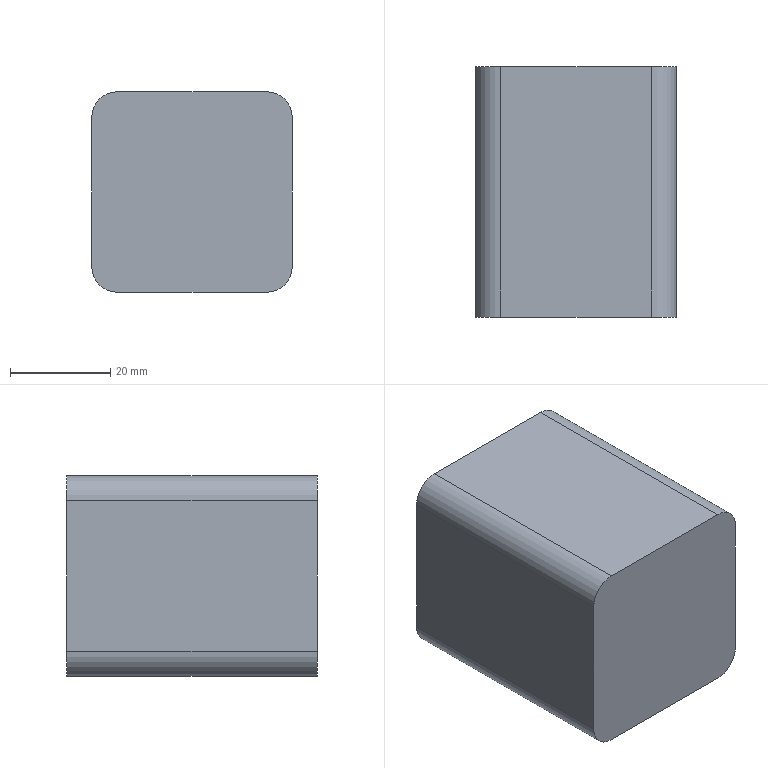Component | SolidWorks | Jig4040-50-5 | 1 solid | 10 faces | box 40 x 50 x 40 mm | volume 78927 mm3 | plane 6 | cylinder 4 | commonest cylinder face diameters 10 x4 | material Copper
build123d program:
from build123d import *

# Parameters (mm, degrees)
BOSS_EXTRUDE1_DEPTH = 50


with BuildPart() as part:
    # Sketch1 → Boss-Extrude1 (new body)
    with BuildSketch(Plane(origin=(0, 0, 0), x_dir=(1, 0, 0), z_dir=(0, 1, 0))):
        with BuildLine():
            Line((5, 0), (35, 0))
            ThreePointArc((35, 0), (38.536, 1.464), (40, 5))
            Line((40, 5), (40, 35))
            ThreePointArc((40, 35), (38.536, 38.536), (35, 40))
            Line((35, 40), (5, 40))
            ThreePointArc((5, 40), (1.464, 38.536), (0, 35))
            Line((0, 35), (0, 5))
            ThreePointArc((0, 5), (1.464, 1.464), (5, 0))
        make_face()
    extrude(amount=BOSS_EXTRUDE1_DEPTH)


solid = part.part

# Placed as in the assembly
solid = solid.moved(Location((711.992, -67.909, 2130), (0, 0, 0)))
STEP:
#1=COLOUR_RGB('',0.7922,0.8196,0.9333);
#2=FILL_AREA_STYLE_COLOUR('',#1);
#3=FILL_AREA_STYLE('',(#2));
#4=SURFACE_STYLE_FILL_AREA(#3);
#5=SURFACE_SIDE_STYLE('',(#4));
#6=SURFACE_STYLE_USAGE(.BOTH.,#5);
#7=PRESENTATION_STYLE_ASSIGNMENT((#6));
#8=CARTESIAN_POINT('',(28.031,-2.674,83.661));
#9=VERTEX_POINT('',#8);
#10=CARTESIAN_POINT('',(28.228,-2.674,83.858));
#11=VERTEX_POINT('',#10);
#12=CARTESIAN_POINT('',(28.228,-2.674,83.661));
#13=DIRECTION('',(0.,1.,0.));
#14=DIRECTION('',(0.,0.,1.));
#15=AXIS2_PLACEMENT_3D('',#12,#13,#14);
#16=CIRCLE('',#15,0.1969);
#17=EDGE_CURVE('',#9,#11,#16,.T.);
#18=ORIENTED_EDGE('',*,*,#17,.T.);
#19=CARTESIAN_POINT('',(28.228,-0.7051,83.858));
#20=VERTEX_POINT('',#19);
#21=CARTESIAN_POINT('',(28.228,-0.7051,83.858));
#22=DIRECTION('',(0.,-1.,0.));
#23=VECTOR('',#22,39.37);
#24=LINE('',#21,#23);
#25=EDGE_CURVE('',#20,#11,#24,.T.);
#26=ORIENTED_EDGE('',*,*,#25,.F.);
#27=CARTESIAN_POINT('',(28.031,-0.7051,83.661));
#28=VERTEX_POINT('',#27);
#29=CARTESIAN_POINT('',(28.228,-0.7051,83.661));
#30=DIRECTION('',(0.,1.,0.));
#31=DIRECTION('',(0.,0.,1.));
#32=AXIS2_PLACEMENT_3D('',#29,#30,#31);
#33=CIRCLE('',#32,0.1969);
#34=EDGE_CURVE('',#28,#20,#33,.T.);
#35=ORIENTED_EDGE('',*,*,#34,.F.);
#36=CARTESIAN_POINT('',(28.031,-0.7051,83.661));
#37=DIRECTION('',(0.,-1.,0.));
#38=VECTOR('',#37,39.37);
#39=LINE('',#36,#38);
#40=EDGE_CURVE('',#28,#9,#39,.T.);
#41=ORIENTED_EDGE('',*,*,#40,.T.);
#42=EDGE_LOOP('',(#18,#26,#35,#41));
#43=FACE_OUTER_BOUND('',#42,.T.);
#44=CARTESIAN_POINT('',(28.228,-0.7051,83.661));
#45=DIRECTION('',(0.,-1.,0.));
#46=DIRECTION('',(0.,0.,-1.));
#47=AXIS2_PLACEMENT_3D('',#44,#45,#46);
#48=CYLINDRICAL_SURFACE('',#47,0.1969);
#49=ADVANCED_FACE('',(#43),#48,.T.);
#50=CARTESIAN_POINT('',(29.409,-2.674,83.858));
#51=VERTEX_POINT('',#50);
#52=CARTESIAN_POINT('',(28.228,-2.674,83.858));
#53=DIRECTION('',(1.,0.,0.));
#54=VECTOR('',#53,39.37);
#55=LINE('',#52,#54);
#56=EDGE_CURVE('',#11,#51,#55,.T.);
#57=ORIENTED_EDGE('',*,*,#56,.T.);
#58=CARTESIAN_POINT('',(29.409,-0.7051,83.858));
#59=VERTEX_POINT('',#58);
#60=CARTESIAN_POINT('',(29.409,-0.7051,83.858));
#61=DIRECTION('',(0.,-1.,0.));
#62=VECTOR('',#61,39.37);
#63=LINE('',#60,#62);
#64=EDGE_CURVE('',#59,#51,#63,.T.);
#65=ORIENTED_EDGE('',*,*,#64,.F.);
#66=CARTESIAN_POINT('',(28.228,-0.7051,83.858));
#67=DIRECTION('',(1.,0.,0.));
#68=VECTOR('',#67,39.37);
#69=LINE('',#66,#68);
#70=EDGE_CURVE('',#20,#59,#69,.T.);
#71=ORIENTED_EDGE('',*,*,#70,.F.);
#72=ORIENTED_EDGE('',*,*,#25,.T.);
#73=EDGE_LOOP('',(#57,#65,#71,#72));
#74=FACE_OUTER_BOUND('',#73,.T.);
#75=CARTESIAN_POINT('',(28.228,-0.7051,83.858));
#76=DIRECTION('',(0.,0.,-1.));
#77=DIRECTION('',(-1.,0.,0.));
#78=AXIS2_PLACEMENT_3D('',#75,#76,#77);
#79=PLANE('',#78);
#80=ADVANCED_FACE('',(#74),#79,.F.);
#81=CARTESIAN_POINT('',(29.606,-2.674,83.661));
#82=VERTEX_POINT('',#81);
#83=CARTESIAN_POINT('',(29.409,-2.674,83.661));
#84=DIRECTION('',(0.,1.,0.));
#85=DIRECTION('',(0.,0.,1.));
#86=AXIS2_PLACEMENT_3D('',#83,#84,#85);
#87=CIRCLE('',#86,0.1969);
#88=EDGE_CURVE('',#51,#82,#87,.T.);
#89=ORIENTED_EDGE('',*,*,#88,.T.);
#90=CARTESIAN_POINT('',(29.606,-0.7051,83.661));
#91=VERTEX_POINT('',#90);
#92=CARTESIAN_POINT('',(29.606,-0.7051,83.661));
#93=DIRECTION('',(0.,-1.,0.));
#94=VECTOR('',#93,39.37);
#95=LINE('',#92,#94);
#96=EDGE_CURVE('',#91,#82,#95,.T.);
#97=ORIENTED_EDGE('',*,*,#96,.F.);
#98=CARTESIAN_POINT('',(29.409,-0.7051,83.661));
#99=DIRECTION('',(0.,1.,0.));
#100=DIRECTION('',(0.,0.,1.));
#101=AXIS2_PLACEMENT_3D('',#98,#99,#100);
#102=CIRCLE('',#101,0.1969);
#103=EDGE_CURVE('',#59,#91,#102,.T.);
#104=ORIENTED_EDGE('',*,*,#103,.F.);
#105=ORIENTED_EDGE('',*,*,#64,.T.);
#106=EDGE_LOOP('',(#89,#97,#104,#105));
#107=FACE_OUTER_BOUND('',#106,.T.);
#108=CARTESIAN_POINT('',(29.409,-0.7051,83.661));
#109=DIRECTION('',(0.,-1.,0.));
#110=DIRECTION('',(0.,0.,-1.));
#111=AXIS2_PLACEMENT_3D('',#108,#109,#110);
#112=CYLINDRICAL_SURFACE('',#111,0.1969);
#113=ADVANCED_FACE('',(#107),#112,.T.);
#114=CARTESIAN_POINT('',(29.606,-2.674,82.48));
#115=VERTEX_POINT('',#114);
#116=CARTESIAN_POINT('',(29.606,-2.674,83.661));
#117=DIRECTION('',(0.,0.,-1.));
#118=VECTOR('',#117,39.37);
#119=LINE('',#116,#118);
#120=EDGE_CURVE('',#82,#115,#119,.T.);
#121=ORIENTED_EDGE('',*,*,#120,.T.);
#122=CARTESIAN_POINT('',(29.606,-0.7051,82.48));
#123=VERTEX_POINT('',#122);
#124=CARTESIAN_POINT('',(29.606,-0.7051,82.48));
#125=DIRECTION('',(0.,-1.,0.));
#126=VECTOR('',#125,39.37);
#127=LINE('',#124,#126);
#128=EDGE_CURVE('',#123,#115,#127,.T.);
#129=ORIENTED_EDGE('',*,*,#128,.F.);
#130=CARTESIAN_POINT('',(29.606,-0.7051,83.661));
#131=DIRECTION('',(0.,0.,-1.));
#132=VECTOR('',#131,39.37);
#133=LINE('',#130,#132);
#134=EDGE_CURVE('',#91,#123,#133,.T.);
#135=ORIENTED_EDGE('',*,*,#134,.F.);
#136=ORIENTED_EDGE('',*,*,#96,.T.);
#137=EDGE_LOOP('',(#121,#129,#135,#136));
#138=FACE_OUTER_BOUND('',#137,.T.);
#139=CARTESIAN_POINT('',(29.606,-0.7051,83.661));
#140=DIRECTION('',(-1.,0.,0.));
#141=DIRECTION('',(0.,0.,1.));
#142=AXIS2_PLACEMENT_3D('',#139,#140,#141);
#143=PLANE('',#142);
#144=ADVANCED_FACE('',(#138),#143,.F.);
#145=CARTESIAN_POINT('',(29.409,-2.674,82.283));
#146=VERTEX_POINT('',#145);
#147=CARTESIAN_POINT('',(29.409,-2.674,82.48));
#148=DIRECTION('',(0.,1.,0.));
#149=DIRECTION('',(0.,0.,-1.));
#150=AXIS2_PLACEMENT_3D('',#147,#148,#149);
#151=CIRCLE('',#150,0.1969);
#152=EDGE_CURVE('',#115,#146,#151,.T.);
#153=ORIENTED_EDGE('',*,*,#152,.T.);
#154=CARTESIAN_POINT('',(29.409,-0.7051,82.283));
#155=VERTEX_POINT('',#154);
#156=CARTESIAN_POINT('',(29.409,-0.7051,82.283));
#157=DIRECTION('',(0.,-1.,0.));
#158=VECTOR('',#157,39.37);
#159=LINE('',#156,#158);
#160=EDGE_CURVE('',#155,#146,#159,.T.);
#161=ORIENTED_EDGE('',*,*,#160,.F.);
#162=CARTESIAN_POINT('',(29.409,-0.7051,82.48));
#163=DIRECTION('',(0.,1.,0.));
#164=DIRECTION('',(0.,0.,-1.));
#165=AXIS2_PLACEMENT_3D('',#162,#163,#164);
#166=CIRCLE('',#165,0.1969);
#167=EDGE_CURVE('',#123,#155,#166,.T.);
#168=ORIENTED_EDGE('',*,*,#167,.F.);
#169=ORIENTED_EDGE('',*,*,#128,.T.);
#170=EDGE_LOOP('',(#153,#161,#168,#169));
#171=FACE_OUTER_BOUND('',#170,.T.);
#172=CARTESIAN_POINT('',(29.409,-0.7051,82.48));
#173=DIRECTION('',(0.,-1.,0.));
#174=DIRECTION('',(0.,0.,-1.));
#175=AXIS2_PLACEMENT_3D('',#172,#173,#174);
#176=CYLINDRICAL_SURFACE('',#175,0.1969);
#177=ADVANCED_FACE('',(#171),#176,.T.);
#178=CARTESIAN_POINT('',(28.228,-2.674,82.283));
#179=VERTEX_POINT('',#178);
#180=CARTESIAN_POINT('',(28.228,-2.674,82.283));
#181=DIRECTION('',(-1.,0.,0.));
#182=VECTOR('',#181,39.37);
#183=LINE('',#180,#182);
#184=EDGE_CURVE('',#146,#179,#183,.T.);
#185=ORIENTED_EDGE('',*,*,#184,.T.);
#186=CARTESIAN_POINT('',(28.228,-0.7051,82.283));
#187=VERTEX_POINT('',#186);
#188=CARTESIAN_POINT('',(28.228,-0.7051,82.283));
#189=DIRECTION('',(0.,-1.,0.));
#190=VECTOR('',#189,39.37);
#191=LINE('',#188,#190);
#192=EDGE_CURVE('',#187,#179,#191,.T.);
#193=ORIENTED_EDGE('',*,*,#192,.F.);
#194=CARTESIAN_POINT('',(28.228,-0.7051,82.283));
#195=DIRECTION('',(-1.,0.,0.));
#196=VECTOR('',#195,39.37);
#197=LINE('',#194,#196);
#198=EDGE_CURVE('',#155,#187,#197,.T.);
#199=ORIENTED_EDGE('',*,*,#198,.F.);
#200=ORIENTED_EDGE('',*,*,#160,.T.);
#201=EDGE_LOOP('',(#185,#193,#199,#200));
#202=FACE_OUTER_BOUND('',#201,.T.);
#203=CARTESIAN_POINT('',(28.228,-0.7051,82.283));
#204=DIRECTION('',(0.,0.,1.));
#205=DIRECTION('',(1.,0.,0.));
#206=AXIS2_PLACEMENT_3D('',#203,#204,#205);
#207=PLANE('',#206);
#208=ADVANCED_FACE('',(#202),#207,.F.);
#209=CARTESIAN_POINT('',(28.031,-2.674,82.48));
#210=VERTEX_POINT('',#209);
#211=CARTESIAN_POINT('',(28.228,-2.674,82.48));
#212=DIRECTION('',(0.,1.,0.));
#213=DIRECTION('',(0.,0.,-1.));
#214=AXIS2_PLACEMENT_3D('',#211,#212,#213);
#215=CIRCLE('',#214,0.1969);
#216=EDGE_CURVE('',#179,#210,#215,.T.);
#217=ORIENTED_EDGE('',*,*,#216,.T.);
#218=CARTESIAN_POINT('',(28.031,-0.7051,82.48));
#219=VERTEX_POINT('',#218);
#220=CARTESIAN_POINT('',(28.031,-0.7051,82.48));
#221=DIRECTION('',(0.,-1.,0.));
#222=VECTOR('',#221,39.37);
#223=LINE('',#220,#222);
#224=EDGE_CURVE('',#219,#210,#223,.T.);
#225=ORIENTED_EDGE('',*,*,#224,.F.);
#226=CARTESIAN_POINT('',(28.228,-0.7051,82.48));
#227=DIRECTION('',(0.,1.,0.));
#228=DIRECTION('',(0.,0.,-1.));
#229=AXIS2_PLACEMENT_3D('',#226,#227,#228);
#230=CIRCLE('',#229,0.1969);
#231=EDGE_CURVE('',#187,#219,#230,.T.);
#232=ORIENTED_EDGE('',*,*,#231,.F.);
#233=ORIENTED_EDGE('',*,*,#192,.T.);
#234=EDGE_LOOP('',(#217,#225,#232,#233));
#235=FACE_OUTER_BOUND('',#234,.T.);
#236=CARTESIAN_POINT('',(28.228,-0.7051,82.48));
#237=DIRECTION('',(0.,-1.,0.));
#238=DIRECTION('',(0.,0.,-1.));
#239=AXIS2_PLACEMENT_3D('',#236,#237,#238);
#240=CYLINDRICAL_SURFACE('',#239,0.1969);
#241=ADVANCED_FACE('',(#235),#240,.T.);
#242=CARTESIAN_POINT('',(28.031,-2.674,83.661));
#243=DIRECTION('',(0.,0.,1.));
#244=VECTOR('',#243,39.37);
#245=LINE('',#242,#244);
#246=EDGE_CURVE('',#210,#9,#245,.T.);
#247=ORIENTED_EDGE('',*,*,#246,.T.);
#248=ORIENTED_EDGE('',*,*,#40,.F.);
#249=CARTESIAN_POINT('',(28.031,-0.7051,83.661));
#250=DIRECTION('',(0.,0.,1.));
#251=VECTOR('',#250,39.37);
#252=LINE('',#249,#251);
#253=EDGE_CURVE('',#219,#28,#252,.T.);
#254=ORIENTED_EDGE('',*,*,#253,.F.);
#255=ORIENTED_EDGE('',*,*,#224,.T.);
#256=EDGE_LOOP('',(#247,#248,#254,#255));
#257=FACE_OUTER_BOUND('',#256,.T.);
#258=CARTESIAN_POINT('',(28.031,-0.7051,83.661));
#259=DIRECTION('',(1.,0.,0.));
#260=DIRECTION('',(0.,0.,-1.));
#261=AXIS2_PLACEMENT_3D('',#258,#259,#260);
#262=PLANE('',#261);
#263=ADVANCED_FACE('',(#257),#262,.F.);
#264=ORIENTED_EDGE('',*,*,#34,.T.);
#265=ORIENTED_EDGE('',*,*,#70,.T.);
#266=ORIENTED_EDGE('',*,*,#103,.T.);
#267=ORIENTED_EDGE('',*,*,#134,.T.);
#268=ORIENTED_EDGE('',*,*,#167,.T.);
#269=ORIENTED_EDGE('',*,*,#198,.T.);
#270=ORIENTED_EDGE('',*,*,#231,.T.);
#271=ORIENTED_EDGE('',*,*,#253,.T.);
#272=EDGE_LOOP('',(#264,#265,#266,#267,#268,#269,#270,#271));
#273=FACE_OUTER_BOUND('',#272,.T.);
#274=CARTESIAN_POINT('',(28.228,-0.7051,83.661));
#275=DIRECTION('',(0.,1.,0.));
#276=DIRECTION('',(0.,0.,1.));
#277=AXIS2_PLACEMENT_3D('',#274,#275,#276);
#278=PLANE('',#277);
#279=ADVANCED_FACE('',(#273),#278,.T.);
#280=ORIENTED_EDGE('',*,*,#17,.F.);
#281=ORIENTED_EDGE('',*,*,#246,.F.);
#282=ORIENTED_EDGE('',*,*,#216,.F.);
#283=ORIENTED_EDGE('',*,*,#184,.F.);
#284=ORIENTED_EDGE('',*,*,#152,.F.);
#285=ORIENTED_EDGE('',*,*,#120,.F.);
#286=ORIENTED_EDGE('',*,*,#88,.F.);
#287=ORIENTED_EDGE('',*,*,#56,.F.);
#288=EDGE_LOOP('',(#280,#281,#282,#283,#284,#285,#286,#287));
#289=FACE_OUTER_BOUND('',#288,.T.);
#290=CARTESIAN_POINT('',(28.228,-2.674,83.661));
#291=DIRECTION('',(0.,1.,0.));
#292=DIRECTION('',(0.,0.,1.));
#293=AXIS2_PLACEMENT_3D('',#290,#291,#292);
#294=PLANE('',#293);
#295=ADVANCED_FACE('',(#289),#294,.F.);
#296=CLOSED_SHELL('',(#49,#80,#113,#144,#177,#208,#241,#263,#279,#295));
#297=MANIFOLD_SOLID_BREP('',#296);
#298=STYLED_ITEM('',(#7),#297);
#299=PRESENTATION_LAYER_ASSIGNMENT('','',(#298));
#300=CARTESIAN_POINT('',(0.,0.,0.));
#301=DIRECTION('',(0.,0.,1.));
#302=DIRECTION('',(1.,0.,0.));
#303=AXIS2_PLACEMENT_3D('',#300,#301,#302);
#304=(LENGTH_UNIT()NAMED_UNIT(*)SI_UNIT($,.METRE.));
#305=LENGTH_MEASURE_WITH_UNIT(LENGTH_MEASURE(0.0254),#304);
#306=DIMENSIONAL_EXPONENTS(1.,0.,0.,0.,0.,0.,0.);
#307=(CONVERSION_BASED_UNIT('',#305)LENGTH_UNIT()NAMED_UNIT(#306));
#308=UNCERTAINTY_MEASURE_WITH_UNIT(LENGTH_MEASURE(0.00001),#307,'','');
#309=(NAMED_UNIT(*)PLANE_ANGLE_UNIT()SI_UNIT($,.RADIAN.));
#310=(NAMED_UNIT(*)SI_UNIT($,.STERADIAN.)SOLID_ANGLE_UNIT());
#311=(GEOMETRIC_REPRESENTATION_CONTEXT(3)GLOBAL_UNCERTAINTY_ASSIGNED_CONTEXT((#308))GLOBAL_UNIT_ASSIGNED_CONTEXT((#307,#309,#310))REPRESENTATION_CONTEXT('',''));
#312=ADVANCED_BREP_SHAPE_REPRESENTATION('',(#297,#303),#311);
#313=(LENGTH_UNIT()NAMED_UNIT(*)SI_UNIT($,.METRE.));
#314=LENGTH_MEASURE_WITH_UNIT(LENGTH_MEASURE(0.0254),#313);
#315=DIMENSIONAL_EXPONENTS(1.,0.,0.,0.,0.,0.,0.);
#316=(CONVERSION_BASED_UNIT('',#314)LENGTH_UNIT()NAMED_UNIT(#315));
#317=UNCERTAINTY_MEASURE_WITH_UNIT(LENGTH_MEASURE(0.00001),#316,'','');
#318=(NAMED_UNIT(*)PLANE_ANGLE_UNIT()SI_UNIT($,.RADIAN.));
#319=(NAMED_UNIT(*)SI_UNIT($,.STERADIAN.)SOLID_ANGLE_UNIT());
#320=(GEOMETRIC_REPRESENTATION_CONTEXT(3)GLOBAL_UNCERTAINTY_ASSIGNED_CONTEXT((#317))GLOBAL_UNIT_ASSIGNED_CONTEXT((#316,#318,#319))REPRESENTATION_CONTEXT('',''));
#321=MECHANICAL_DESIGN_GEOMETRIC_PRESENTATION_REPRESENTATION('',(#298),#320);